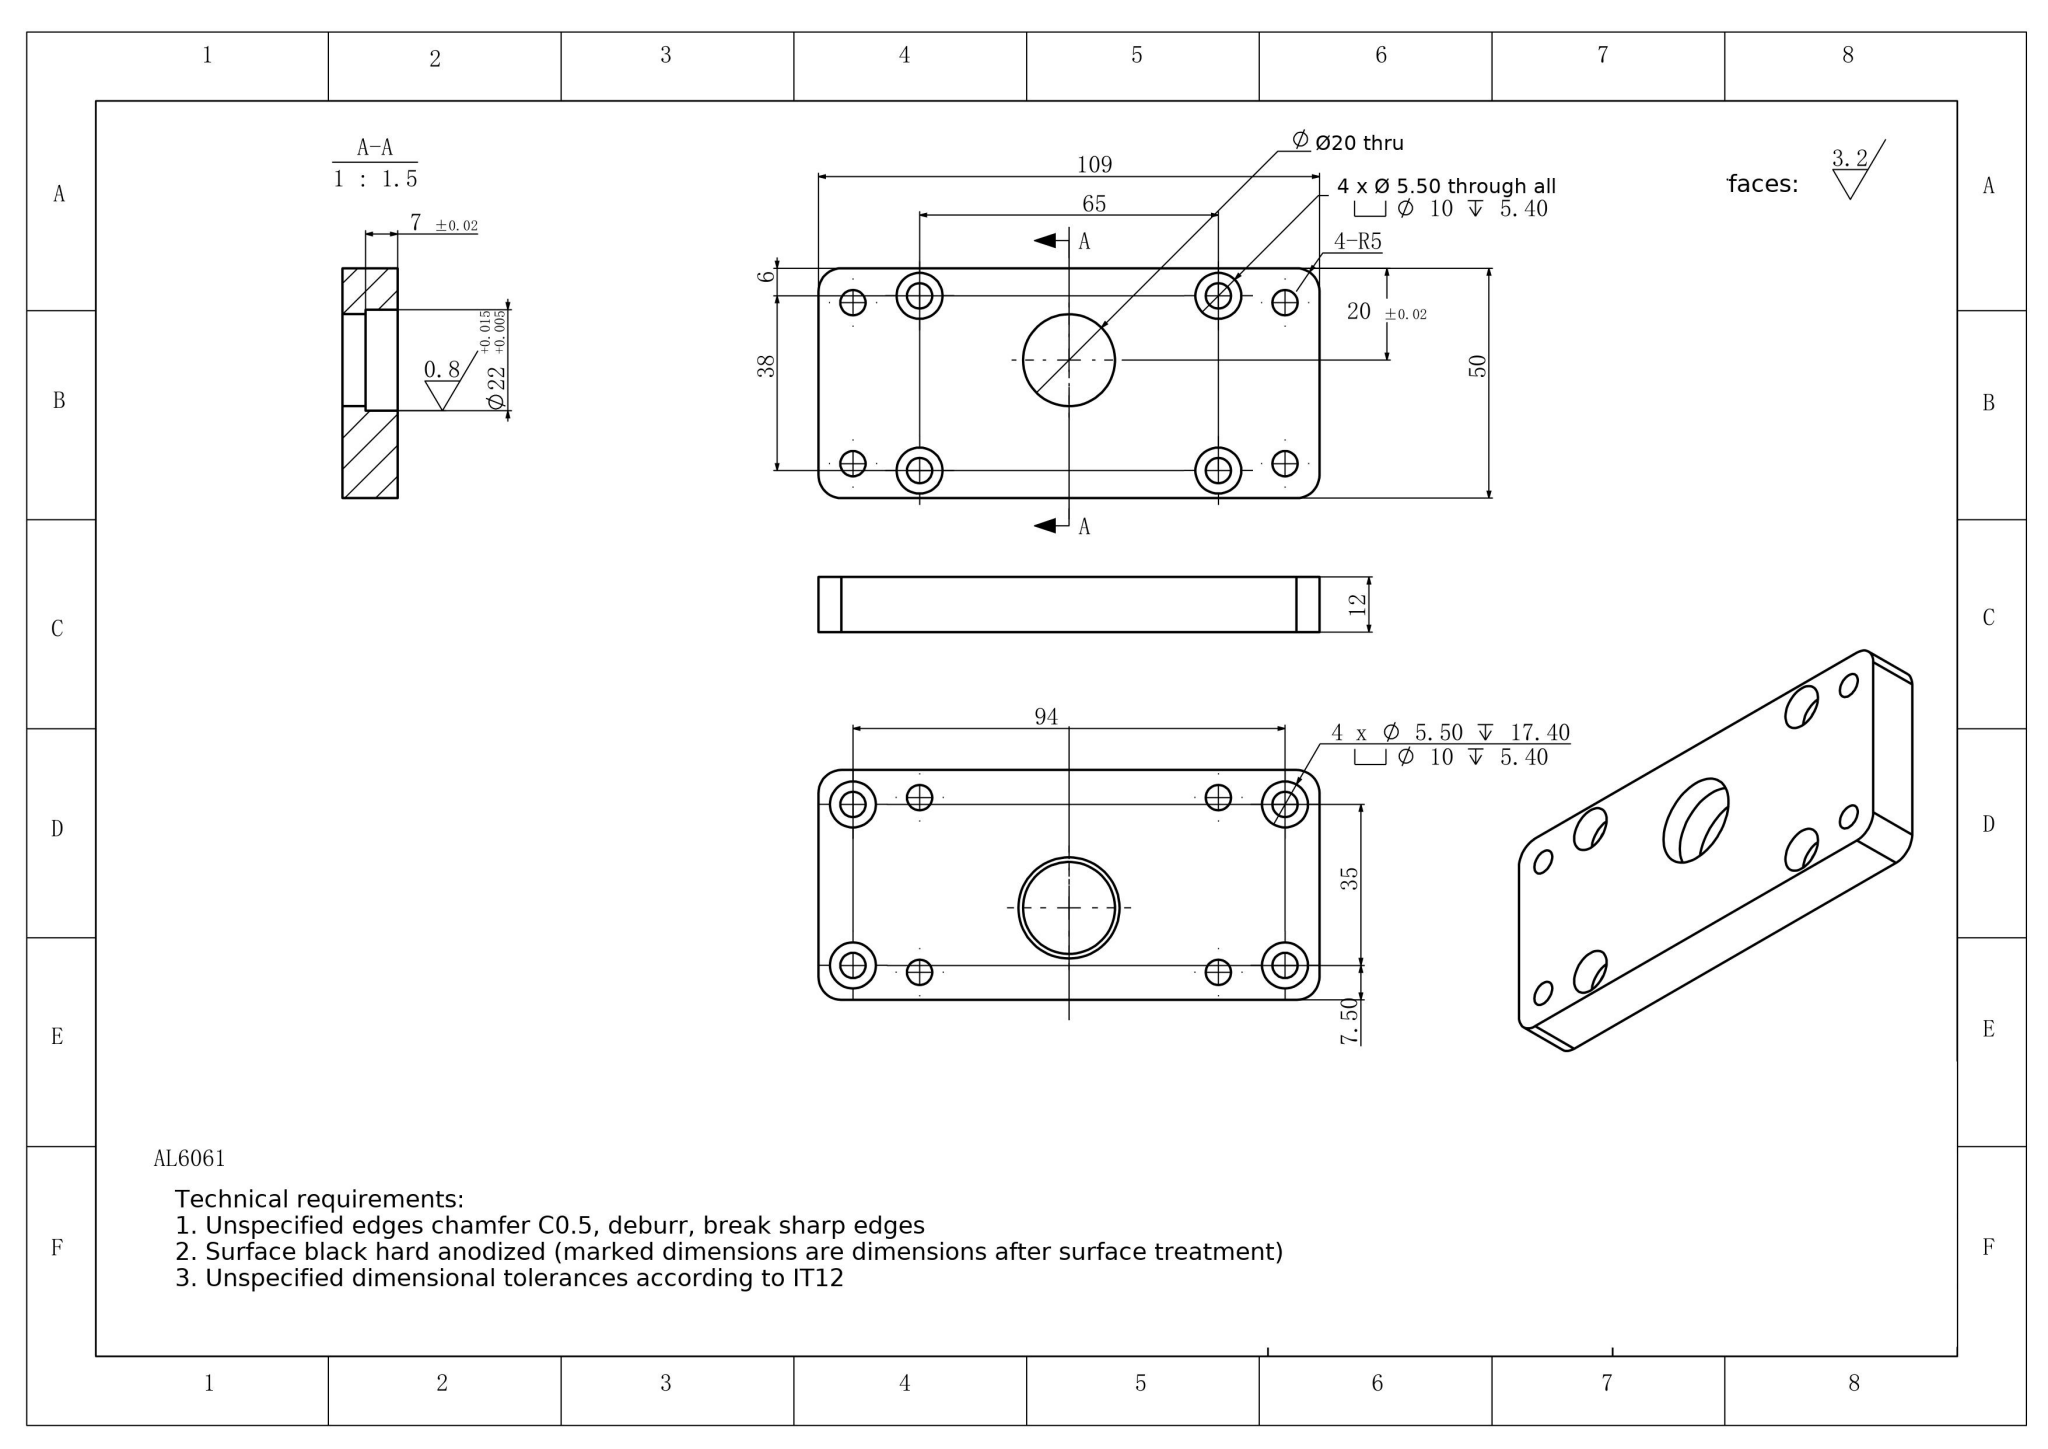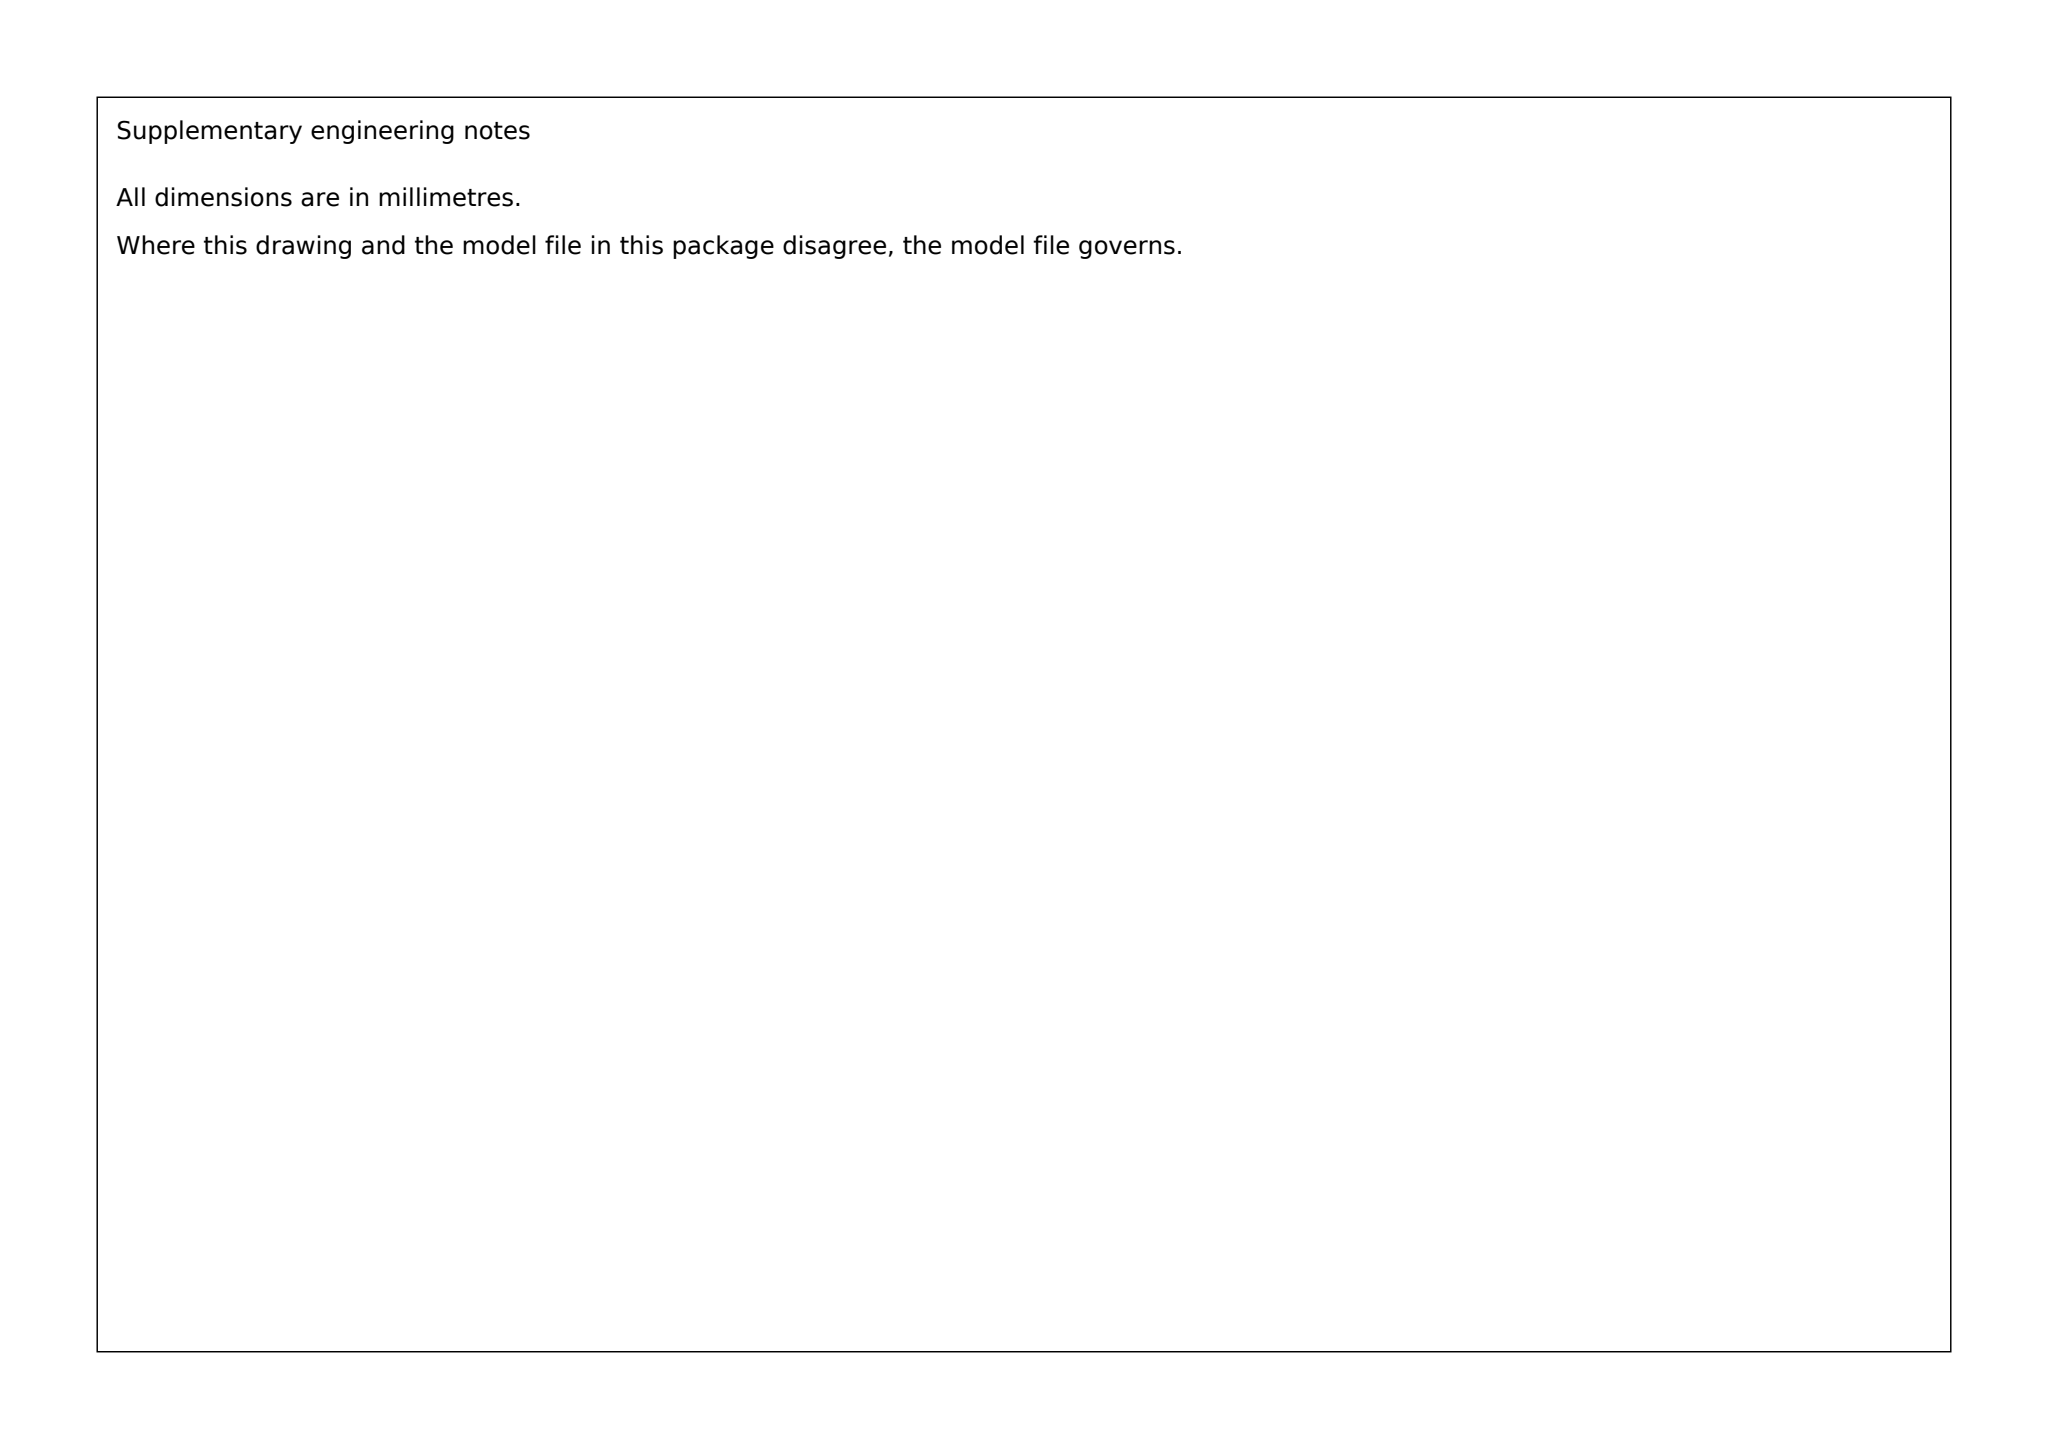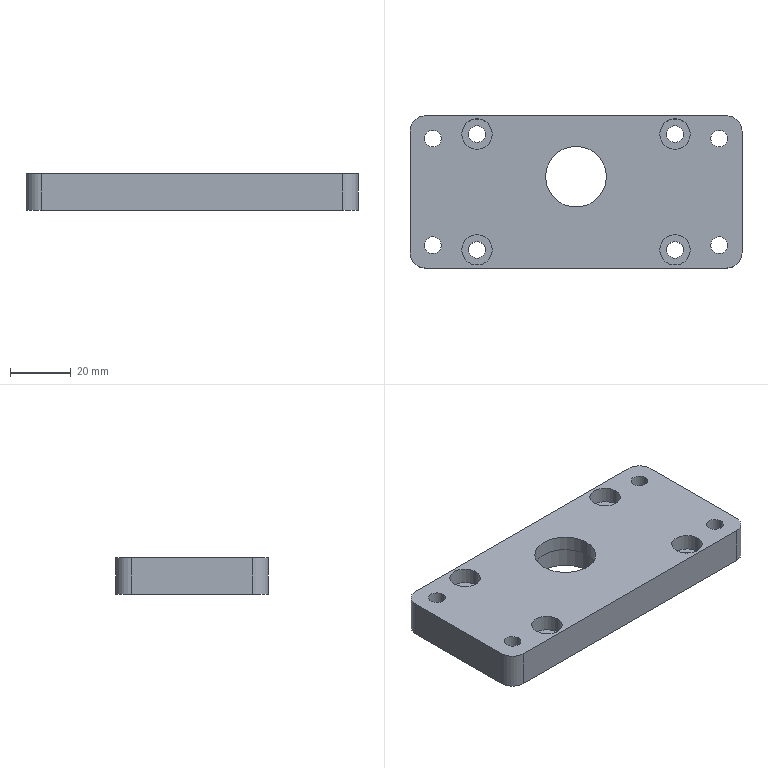Part | SolidWorks | mm | material AL6061 | 1 solid | 55 faces | box 109 x 50 x 12 mm | volume 56263 mm3 | cylinder 40 | plane 15 | commonest cylinder face diameters 10 x20 5.5 x16 20 x2 22 x2
build123d program:
from build123d import *

# Parameters (mm, degrees)
SKETCH1_W                                       = 77
SKETCH1_H                                       = 50
BOSS_EXTRUDE1_DEPTH                             = 12
M5_HEX_SOCKET_HEAD_CAP_SCREW_CBORE1_D           = 5.5
M5_HEX_SOCKET_HEAD_CAP_SCREW_CBORE1_CBORE_D     = 10
M5_HEX_SOCKET_HEAD_CAP_SCREW_CBORE1_CBORE_DEPTH = 5.4
SKETCH4_R                                       = 11
CUT_EXTRUDE1_DEPTH                              = 7
SKETCH5_R                                       = 10
CUT_EXTRUDE2_DEPTH                              = 47.435
SKETCH6_W                                       = 16
SKETCH6_H                                       = 50
BOSS_EXTRUDE2_DEPTH                             = 12
M5_HEX_SOCKET_HEAD_CAP_SCREW_CBORE2_D           = 5.5
M5_HEX_SOCKET_HEAD_CAP_SCREW_CBORE2_DEPTH       = 17.4
M5_HEX_SOCKET_HEAD_CAP_SCREW_CBORE2_CBORE_D     = 10
M5_HEX_SOCKET_HEAD_CAP_SCREW_CBORE2_CBORE_DEPTH = 5.4
M5_HEX_SOCKET_HEAD_CAP_SCREW_CBORE2_TIP         = 1.652
FILLET2_R                                       = 5


with BuildPart() as part:
    # Sketch1 → Boss-Extrude1 (new body)
    with BuildSketch(Plane.XY):
        Rectangle(SKETCH1_W, SKETCH1_H)
    extrude(amount=BOSS_EXTRUDE1_DEPTH)

    # M5 Hex Socket Head Cap Screw CBORE1 (through all)
    with Locations(Plane.XY.offset(12)):
        with Locations((-32.5, 19), (-32.5, -19), (32.5, 19), (32.5, -19)):
            CounterBoreHole(M5_HEX_SOCKET_HEAD_CAP_SCREW_CBORE1_D / 2, M5_HEX_SOCKET_HEAD_CAP_SCREW_CBORE1_CBORE_D / 2, M5_HEX_SOCKET_HEAD_CAP_SCREW_CBORE1_CBORE_DEPTH)

    # Sketch4 → Cut-Extrude1 (cut)
    with BuildSketch(Plane(origin=(0, 0, 0), x_dir=(-1, 0, 0), z_dir=(0, 0, -1))):
        with Locations((0, 5)):
            Circle(SKETCH4_R)
    extrude(amount=-CUT_EXTRUDE1_DEPTH, mode=Mode.SUBTRACT)

    # Sketch5 → Cut-Extrude2 (cut, through all)
    with BuildSketch(Plane(origin=(0, 0, 7), x_dir=(-1, 0, 0), z_dir=(0, 0, -1))):
        with Locations((0, 5)):
            Circle(SKETCH5_R)
    extrude(amount=-CUT_EXTRUDE2_DEPTH, mode=Mode.SUBTRACT)

    # Sketch6 → Boss-Extrude2 (add)
    with BuildSketch(Plane(origin=(0, 0, 0), x_dir=(-1, 0, 0), z_dir=(0, 0, -1))):
        with Locations((46.5, 0)):
            Rectangle(SKETCH6_W, SKETCH6_H)
        with Locations((-46.5, 0)):
            Rectangle(SKETCH6_W, SKETCH6_H)
    extrude(amount=-BOSS_EXTRUDE2_DEPTH)

    # M5 Hex Socket Head Cap Screw CBORE2
    with Locations(Plane(origin=(0, 0, 0), x_dir=(-1, 0, 0), z_dir=(0, 0, -1))):
        with Locations((47, -17.5), (47, 17.5), (-47, -17.5), (-47, 17.5)):
            CounterBoreHole(M5_HEX_SOCKET_HEAD_CAP_SCREW_CBORE2_D / 2, M5_HEX_SOCKET_HEAD_CAP_SCREW_CBORE2_CBORE_D / 2, M5_HEX_SOCKET_HEAD_CAP_SCREW_CBORE2_CBORE_DEPTH, depth=M5_HEX_SOCKET_HEAD_CAP_SCREW_CBORE2_DEPTH)
            with Locations((0, 0, -(M5_HEX_SOCKET_HEAD_CAP_SCREW_CBORE2_DEPTH + M5_HEX_SOCKET_HEAD_CAP_SCREW_CBORE2_TIP / 2))):  # 118° drill point
                Cone(0, M5_HEX_SOCKET_HEAD_CAP_SCREW_CBORE2_D / 2, M5_HEX_SOCKET_HEAD_CAP_SCREW_CBORE2_TIP, mode=Mode.SUBTRACT)

    # Fillet2
    fillet2_edges = [part.edges().sort_by_distance(p)[0] for p in [
        (-54.5, 25, 6),
        (-54.5, -25, 6),
        (54.5, -25, 6),
        (54.5, 25, 6),
    ]]
    fillet(fillet2_edges, radius=FILLET2_R)


solid = part.part